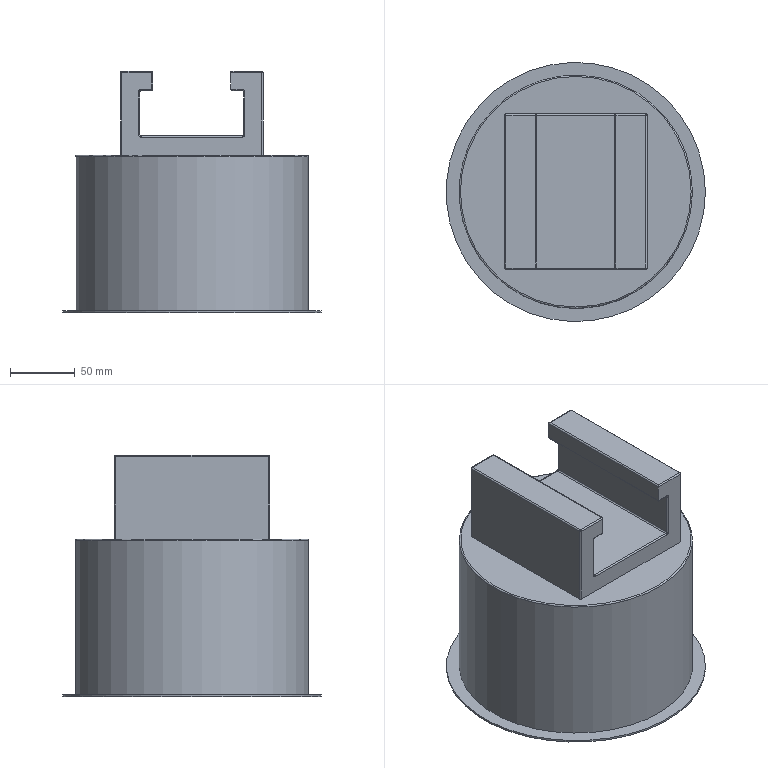Component | NX | A_PART_2 | 1 solid | 65 faces | volume 3514425 mm3 | cylinder 32 | plane 16 | torus 9 | sphere 8 | commonest cylinder face diameters 2 x30 180 x1 200 x1